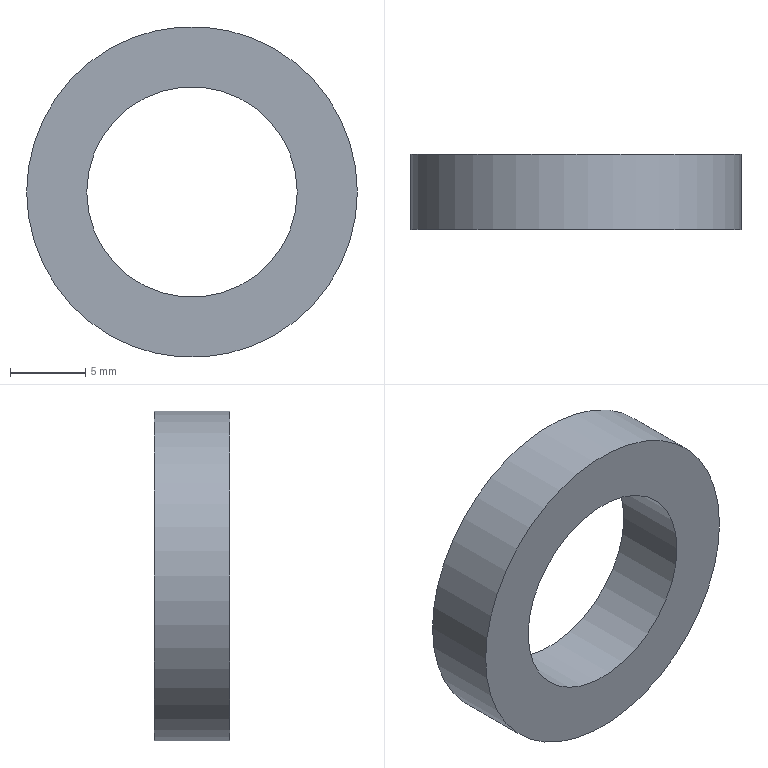Component | NX | SEAL_RING | 1 solid | 4 faces | box 22 x 5 x 22 mm | volume 1131 mm3 | cylinder 2 | plane 2 | commonest cylinder face diameters 22 x1 14 x1
STEP:
#1=CARTESIAN_POINT('',(0.,0.,0.));
#2=DIRECTION('',(0.,0.,1.));
#3=DIRECTION('',(1.,0.,0.));
#4=AXIS2_PLACEMENT_3D('',#1,#2,#3);
#5=CARTESIAN_POINT('',(11.,29.,4.5));
#6=VERTEX_POINT('',#5);
#7=CARTESIAN_POINT('',(-0.,29.,4.5));
#8=DIRECTION('',(0.,-1.,0.));
#9=DIRECTION('',(1.,0.,-0.));
#10=AXIS2_PLACEMENT_3D('',#7,#8,#9);
#11=CIRCLE('',#10,11.);
#12=CARTESIAN_POINT('',(-0.,35.,4.5));
#13=DIRECTION('',(0.,-1.,0.));
#14=DIRECTION('',(-1.,0.,0.));
#15=AXIS2_PLACEMENT_3D('',#12,#13,#14);
#16=CYLINDRICAL_SURFACE('',#15,11.);
#17=CARTESIAN_POINT('',(3.142,6.));
#18=DIRECTION('',(1.,0.));
#19=VECTOR('',#18,1.);
#20=LINE('',#17,#19);
#21=(GEOMETRIC_REPRESENTATION_CONTEXT(2)PARAMETRIC_REPRESENTATION_CONTEXT()REPRESENTATION_CONTEXT('',''));
#22=DEFINITIONAL_REPRESENTATION('',(#20),#21);
#23=PCURVE('',#16,#22);
#24=CARTESIAN_POINT('',(-0.,29.,4.5));
#25=DIRECTION('',(0.,-1.,0.));
#26=DIRECTION('',(-1.,0.,0.));
#27=AXIS2_PLACEMENT_3D('',#24,#25,#26);
#28=PLANE('',#27);
#29=CARTESIAN_POINT('',(0.,0.));
#30=DIRECTION('',(-1.,0.));
#31=AXIS2_PLACEMENT_2D('',#29,#30);
#32=CIRCLE('',#31,11.);
#33=(GEOMETRIC_REPRESENTATION_CONTEXT(2)PARAMETRIC_REPRESENTATION_CONTEXT()REPRESENTATION_CONTEXT('',''));
#34=DEFINITIONAL_REPRESENTATION('',(#32),#33);
#35=PCURVE('',#28,#34);
#36=SURFACE_CURVE('',#11,(#23,#35),.PCURVE_S1.);
#37=EDGE_CURVE('',#6,#6,#36,.T.);
#38=ORIENTED_EDGE('',*,*,#37,.F.);
#39=CARTESIAN_POINT('',(11.,34.,4.5));
#40=VERTEX_POINT('',#39);
#41=CARTESIAN_POINT('',(11.,34.,4.5));
#42=CARTESIAN_POINT('',(11.,29.,4.5));
#43=B_SPLINE_CURVE_WITH_KNOTS('',1,(#41,#42),.UNSPECIFIED.,.F.,.F.,(2,2),(1.,6.),.PIECEWISE_BEZIER_KNOTS.);
#44=CARTESIAN_POINT('',(3.142,0.));
#45=DIRECTION('',(0.,1.));
#46=VECTOR('',#45,1.);
#47=LINE('',#44,#46);
#48=(GEOMETRIC_REPRESENTATION_CONTEXT(2)PARAMETRIC_REPRESENTATION_CONTEXT()REPRESENTATION_CONTEXT('',''));
#49=DEFINITIONAL_REPRESENTATION('',(#47),#48);
#50=PCURVE('',#16,#49);
#51=CARTESIAN_POINT('',(9.425,0.));
#52=DIRECTION('',(0.,1.));
#53=VECTOR('',#52,1.);
#54=LINE('',#51,#53);
#55=(GEOMETRIC_REPRESENTATION_CONTEXT(2)PARAMETRIC_REPRESENTATION_CONTEXT()REPRESENTATION_CONTEXT('',''));
#56=DEFINITIONAL_REPRESENTATION('',(#54),#55);
#57=PCURVE('',#16,#56);
#58=SEAM_CURVE('',#43,(#50,#57),.PCURVE_S1.);
#59=EDGE_CURVE('',#40,#6,#58,.T.);
#60=ORIENTED_EDGE('',*,*,#59,.F.);
#61=CARTESIAN_POINT('',(-0.,34.,4.5));
#62=DIRECTION('',(0.,-1.,0.));
#63=DIRECTION('',(1.,0.,0.));
#64=AXIS2_PLACEMENT_3D('',#61,#62,#63);
#65=CIRCLE('',#64,11.);
#66=CARTESIAN_POINT('',(3.142,1.));
#67=DIRECTION('',(1.,0.));
#68=VECTOR('',#67,1.);
#69=LINE('',#66,#68);
#70=(GEOMETRIC_REPRESENTATION_CONTEXT(2)PARAMETRIC_REPRESENTATION_CONTEXT()REPRESENTATION_CONTEXT('',''));
#71=DEFINITIONAL_REPRESENTATION('',(#69),#70);
#72=PCURVE('',#16,#71);
#73=CARTESIAN_POINT('',(-0.,34.,4.5));
#74=DIRECTION('',(0.,1.,0.));
#75=DIRECTION('',(1.,0.,0.));
#76=AXIS2_PLACEMENT_3D('',#73,#74,#75);
#77=PLANE('',#76);
#78=CARTESIAN_POINT('',(11.,0.));
#79=CARTESIAN_POINT('',(11.,-19.053));
#80=CARTESIAN_POINT('',(-5.5,-9.526));
#81=CARTESIAN_POINT('',(-22.,-0.));
#82=CARTESIAN_POINT('',(-5.5,9.526));
#83=CARTESIAN_POINT('',(11.,19.053));
#84=CARTESIAN_POINT('',(11.,0.));
#85=(BOUNDED_CURVE()B_SPLINE_CURVE(2,(#78,#79,#80,#81,#82,#83,#84),.UNSPECIFIED.,.T.,.F.)B_SPLINE_CURVE_WITH_KNOTS((1,2,2,2,2,1),(-2.094,0.,2.094,4.189,6.283,8.378),.UNSPECIFIED.)CURVE()GEOMETRIC_REPRESENTATION_ITEM()RATIONAL_B_SPLINE_CURVE((1.,0.5,1.,0.5,1.,0.5,1.))REPRESENTATION_ITEM(''));
#86=(GEOMETRIC_REPRESENTATION_CONTEXT(2)PARAMETRIC_REPRESENTATION_CONTEXT()REPRESENTATION_CONTEXT('',''));
#87=DEFINITIONAL_REPRESENTATION('',(#85),#86);
#88=PCURVE('',#77,#87);
#89=SURFACE_CURVE('',#65,(#72,#88),.PCURVE_S1.);
#90=EDGE_CURVE('',#40,#40,#89,.T.);
#91=ORIENTED_EDGE('',*,*,#90,.T.);
#92=ORIENTED_EDGE('',*,*,#59,.T.);
#93=EDGE_LOOP('',(#38,#60,#91,#92));
#94=FACE_BOUND('',#93,.T.);
#95=ADVANCED_FACE('',(#94),#16,.T.);
#96=CARTESIAN_POINT('',(7.,29.,4.5));
#97=VERTEX_POINT('',#96);
#98=CARTESIAN_POINT('',(-0.,29.,4.5));
#99=DIRECTION('',(0.,-1.,0.));
#100=DIRECTION('',(1.,0.,-0.));
#101=AXIS2_PLACEMENT_3D('',#98,#99,#100);
#102=CIRCLE('',#101,7.);
#103=CARTESIAN_POINT('',(-0.,35.,4.5));
#104=DIRECTION('',(0.,-1.,0.));
#105=DIRECTION('',(-1.,0.,0.));
#106=AXIS2_PLACEMENT_3D('',#103,#104,#105);
#107=CYLINDRICAL_SURFACE('',#106,7.);
#108=CARTESIAN_POINT('',(3.142,6.));
#109=DIRECTION('',(1.,0.));
#110=VECTOR('',#109,1.);
#111=LINE('',#108,#110);
#112=(GEOMETRIC_REPRESENTATION_CONTEXT(2)PARAMETRIC_REPRESENTATION_CONTEXT()REPRESENTATION_CONTEXT('',''));
#113=DEFINITIONAL_REPRESENTATION('',(#111),#112);
#114=PCURVE('',#107,#113);
#115=CARTESIAN_POINT('',(0.,0.));
#116=DIRECTION('',(-1.,0.));
#117=AXIS2_PLACEMENT_2D('',#115,#116);
#118=CIRCLE('',#117,7.);
#119=(GEOMETRIC_REPRESENTATION_CONTEXT(2)PARAMETRIC_REPRESENTATION_CONTEXT()REPRESENTATION_CONTEXT('',''));
#120=DEFINITIONAL_REPRESENTATION('',(#118),#119);
#121=PCURVE('',#28,#120);
#122=SURFACE_CURVE('',#102,(#114,#121),.PCURVE_S1.);
#123=EDGE_CURVE('',#97,#97,#122,.T.);
#124=ORIENTED_EDGE('',*,*,#123,.F.);
#125=CARTESIAN_POINT('',(7.,34.,4.5));
#126=VERTEX_POINT('',#125);
#127=CARTESIAN_POINT('',(7.,34.,4.5));
#128=CARTESIAN_POINT('',(7.,29.,4.5));
#129=B_SPLINE_CURVE_WITH_KNOTS('',1,(#127,#128),.UNSPECIFIED.,.F.,.F.,(2,2),(1.,6.),.PIECEWISE_BEZIER_KNOTS.);
#130=CARTESIAN_POINT('',(3.142,0.));
#131=DIRECTION('',(0.,1.));
#132=VECTOR('',#131,1.);
#133=LINE('',#130,#132);
#134=(GEOMETRIC_REPRESENTATION_CONTEXT(2)PARAMETRIC_REPRESENTATION_CONTEXT()REPRESENTATION_CONTEXT('',''));
#135=DEFINITIONAL_REPRESENTATION('',(#133),#134);
#136=PCURVE('',#107,#135);
#137=CARTESIAN_POINT('',(9.425,0.));
#138=DIRECTION('',(0.,1.));
#139=VECTOR('',#138,1.);
#140=LINE('',#137,#139);
#141=(GEOMETRIC_REPRESENTATION_CONTEXT(2)PARAMETRIC_REPRESENTATION_CONTEXT()REPRESENTATION_CONTEXT('',''));
#142=DEFINITIONAL_REPRESENTATION('',(#140),#141);
#143=PCURVE('',#107,#142);
#144=SEAM_CURVE('',#129,(#136,#143),.PCURVE_S1.);
#145=EDGE_CURVE('',#126,#97,#144,.T.);
#146=ORIENTED_EDGE('',*,*,#145,.F.);
#147=CARTESIAN_POINT('',(-0.,34.,4.5));
#148=DIRECTION('',(0.,-1.,0.));
#149=DIRECTION('',(1.,0.,0.));
#150=AXIS2_PLACEMENT_3D('',#147,#148,#149);
#151=CIRCLE('',#150,7.);
#152=CARTESIAN_POINT('',(3.142,1.));
#153=DIRECTION('',(1.,0.));
#154=VECTOR('',#153,1.);
#155=LINE('',#152,#154);
#156=(GEOMETRIC_REPRESENTATION_CONTEXT(2)PARAMETRIC_REPRESENTATION_CONTEXT()REPRESENTATION_CONTEXT('',''));
#157=DEFINITIONAL_REPRESENTATION('',(#155),#156);
#158=PCURVE('',#107,#157);
#159=CARTESIAN_POINT('',(7.,0.));
#160=CARTESIAN_POINT('',(7.,-12.124));
#161=CARTESIAN_POINT('',(-3.5,-6.062));
#162=CARTESIAN_POINT('',(-14.,-0.));
#163=CARTESIAN_POINT('',(-3.5,6.062));
#164=CARTESIAN_POINT('',(7.,12.124));
#165=CARTESIAN_POINT('',(7.,0.));
#166=(BOUNDED_CURVE()B_SPLINE_CURVE(2,(#159,#160,#161,#162,#163,#164,#165),.UNSPECIFIED.,.T.,.F.)B_SPLINE_CURVE_WITH_KNOTS((1,2,2,2,2,1),(-2.094,0.,2.094,4.189,6.283,8.378),.UNSPECIFIED.)CURVE()GEOMETRIC_REPRESENTATION_ITEM()RATIONAL_B_SPLINE_CURVE((1.,0.5,1.,0.5,1.,0.5,1.))REPRESENTATION_ITEM(''));
#167=(GEOMETRIC_REPRESENTATION_CONTEXT(2)PARAMETRIC_REPRESENTATION_CONTEXT()REPRESENTATION_CONTEXT('',''));
#168=DEFINITIONAL_REPRESENTATION('',(#166),#167);
#169=PCURVE('',#77,#168);
#170=SURFACE_CURVE('',#151,(#158,#169),.PCURVE_S1.);
#171=EDGE_CURVE('',#126,#126,#170,.T.);
#172=ORIENTED_EDGE('',*,*,#171,.T.);
#173=ORIENTED_EDGE('',*,*,#145,.T.);
#174=EDGE_LOOP('',(#124,#146,#172,#173));
#175=FACE_BOUND('',#174,.F.);
#176=ADVANCED_FACE('',(#175),#107,.F.);
#177=ORIENTED_EDGE('',*,*,#37,.T.);
#178=EDGE_LOOP('',(#177));
#179=FACE_BOUND('',#178,.T.);
#180=ORIENTED_EDGE('',*,*,#123,.F.);
#181=EDGE_LOOP('',(#180));
#182=FACE_BOUND('',#181,.T.);
#183=ADVANCED_FACE('',(#179,#182),#28,.T.);
#184=ORIENTED_EDGE('',*,*,#90,.F.);
#185=EDGE_LOOP('',(#184));
#186=FACE_BOUND('',#185,.T.);
#187=ORIENTED_EDGE('',*,*,#171,.T.);
#188=EDGE_LOOP('',(#187));
#189=FACE_BOUND('',#188,.T.);
#190=ADVANCED_FACE('',(#186,#189),#77,.T.);
#191=CLOSED_SHELL('',(#95,#176,#183,#190));
#192=MANIFOLD_SOLID_BREP('',#191);
#193=(LENGTH_UNIT()NAMED_UNIT(*)SI_UNIT(.MILLI.,.METRE.));
#194=UNCERTAINTY_MEASURE_WITH_UNIT(LENGTH_MEASURE(0.00001),#193,'','');
#195=(NAMED_UNIT(*)PLANE_ANGLE_UNIT()SI_UNIT($,.RADIAN.));
#196=(NAMED_UNIT(*)SI_UNIT($,.STERADIAN.)SOLID_ANGLE_UNIT());
#197=(GEOMETRIC_REPRESENTATION_CONTEXT(3)GLOBAL_UNCERTAINTY_ASSIGNED_CONTEXT((#194))GLOBAL_UNIT_ASSIGNED_CONTEXT((#193,#195,#196))REPRESENTATION_CONTEXT('',''));
#198=ADVANCED_BREP_SHAPE_REPRESENTATION('',(#4,#192),#197);